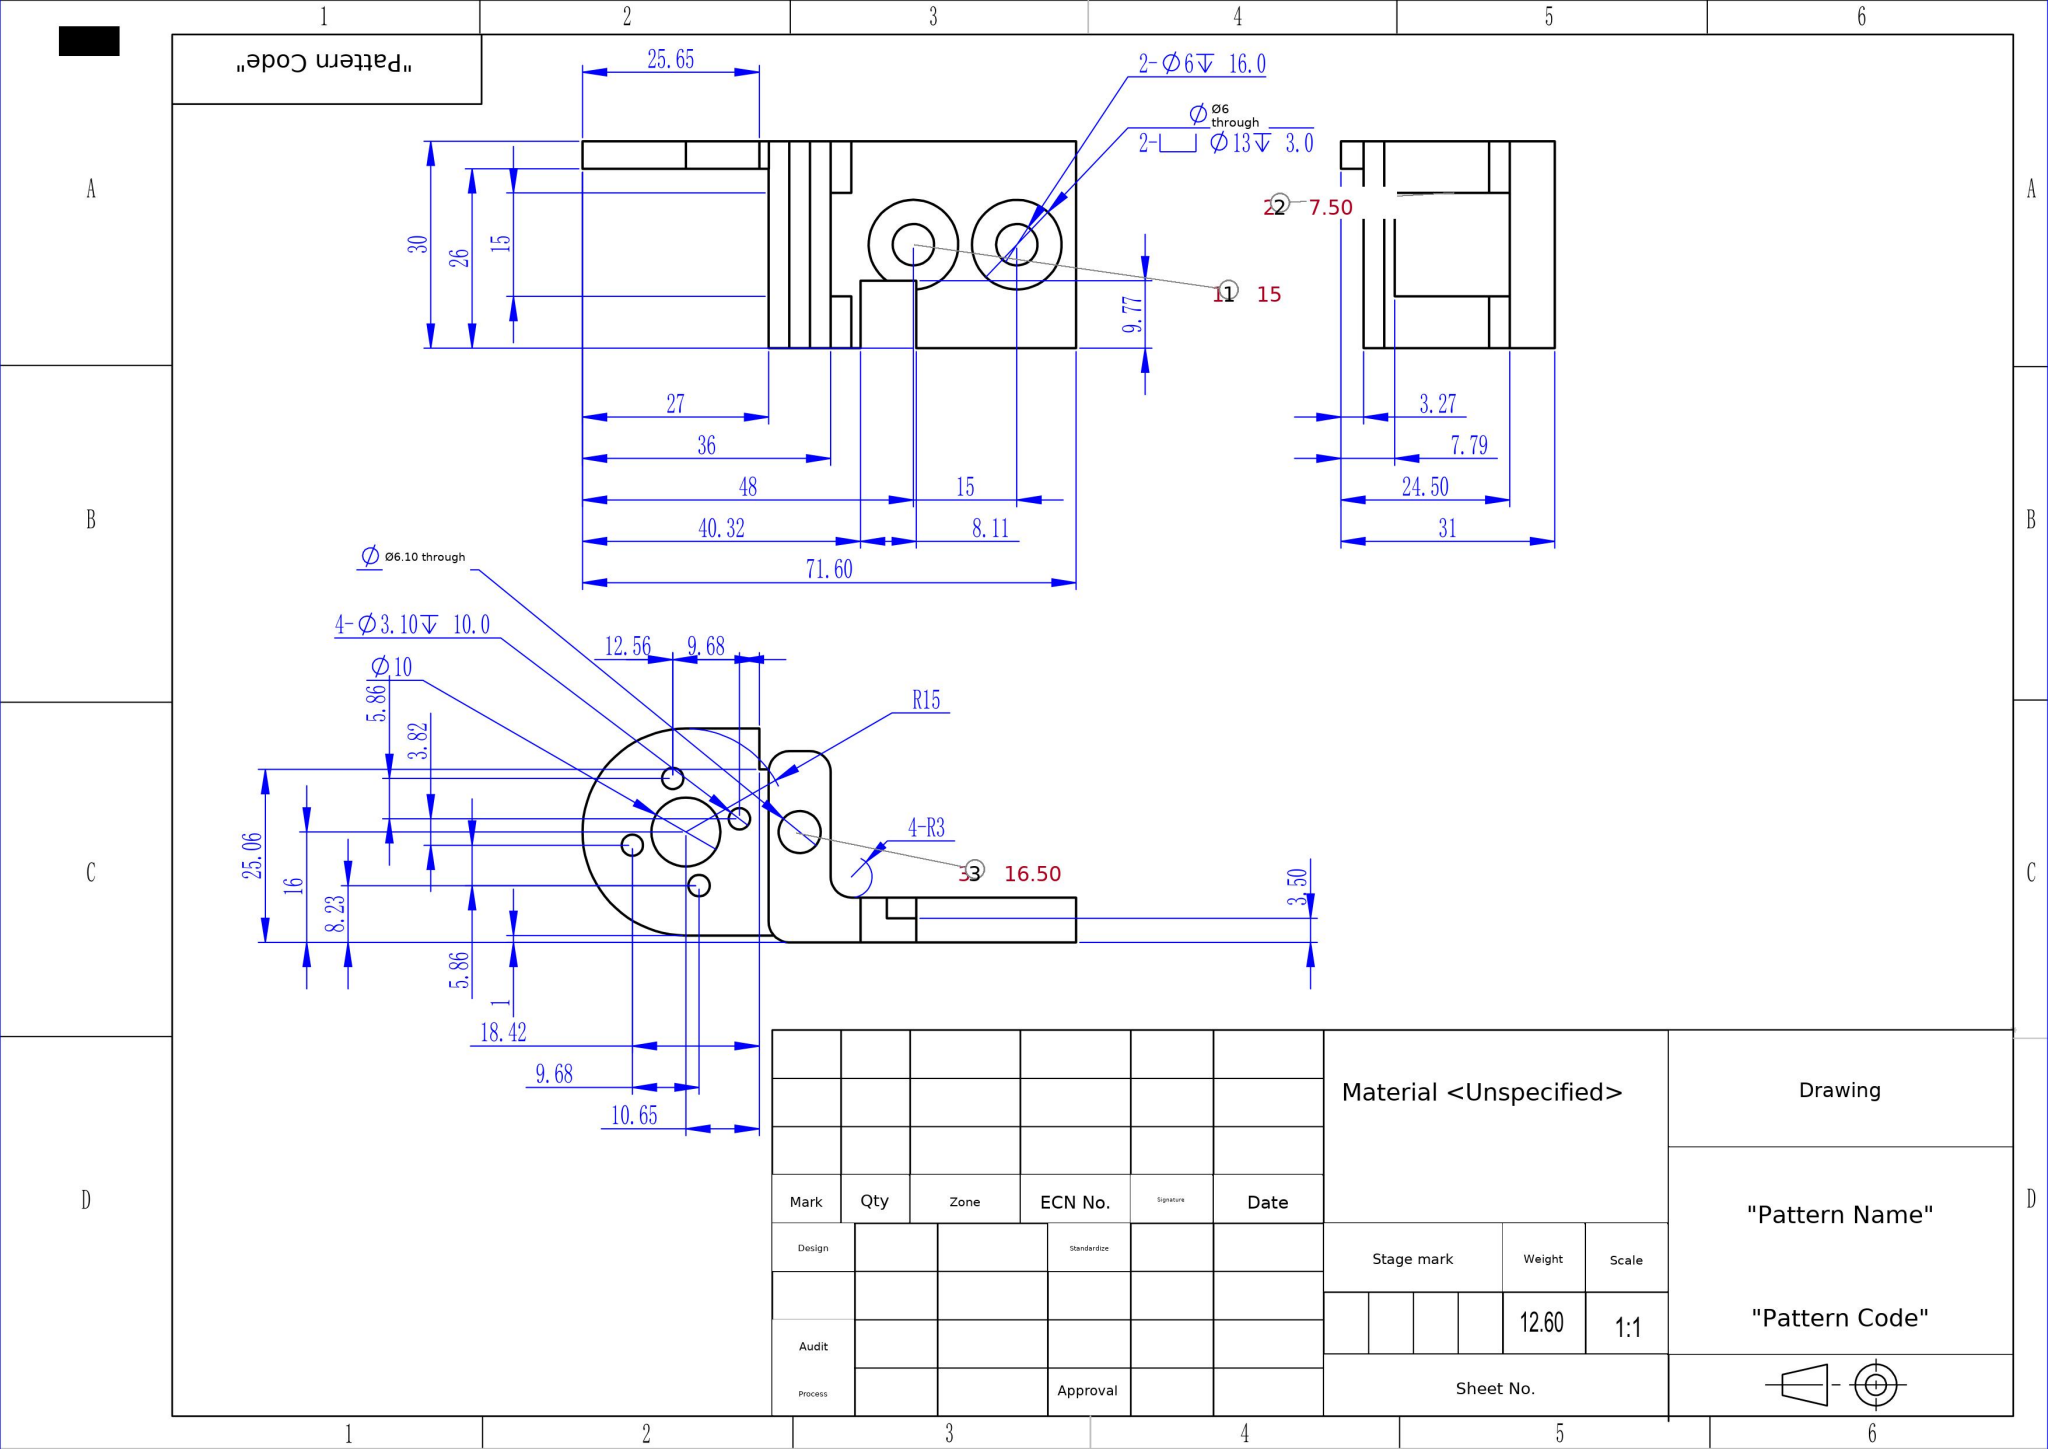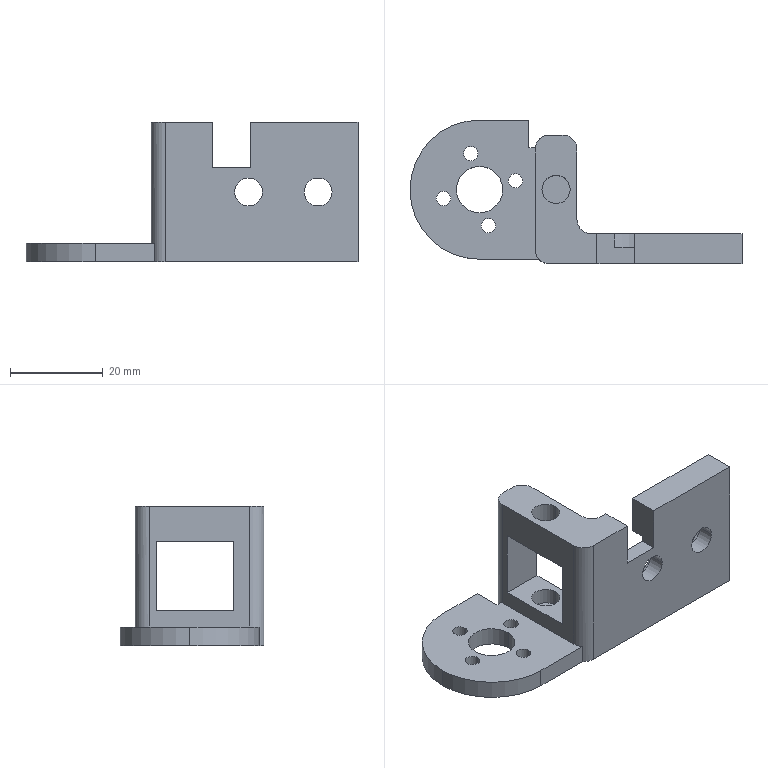Part | SolidWorks | mm | 1 solid | 53 faces | box 71.6 x 31 x 30 mm | volume 12598 mm3 | cylinder 30 | plane 23 | commonest cylinder face diameters 6 x9 3.1 x8 13 x5 6.1 x4 10 x2 30 x2